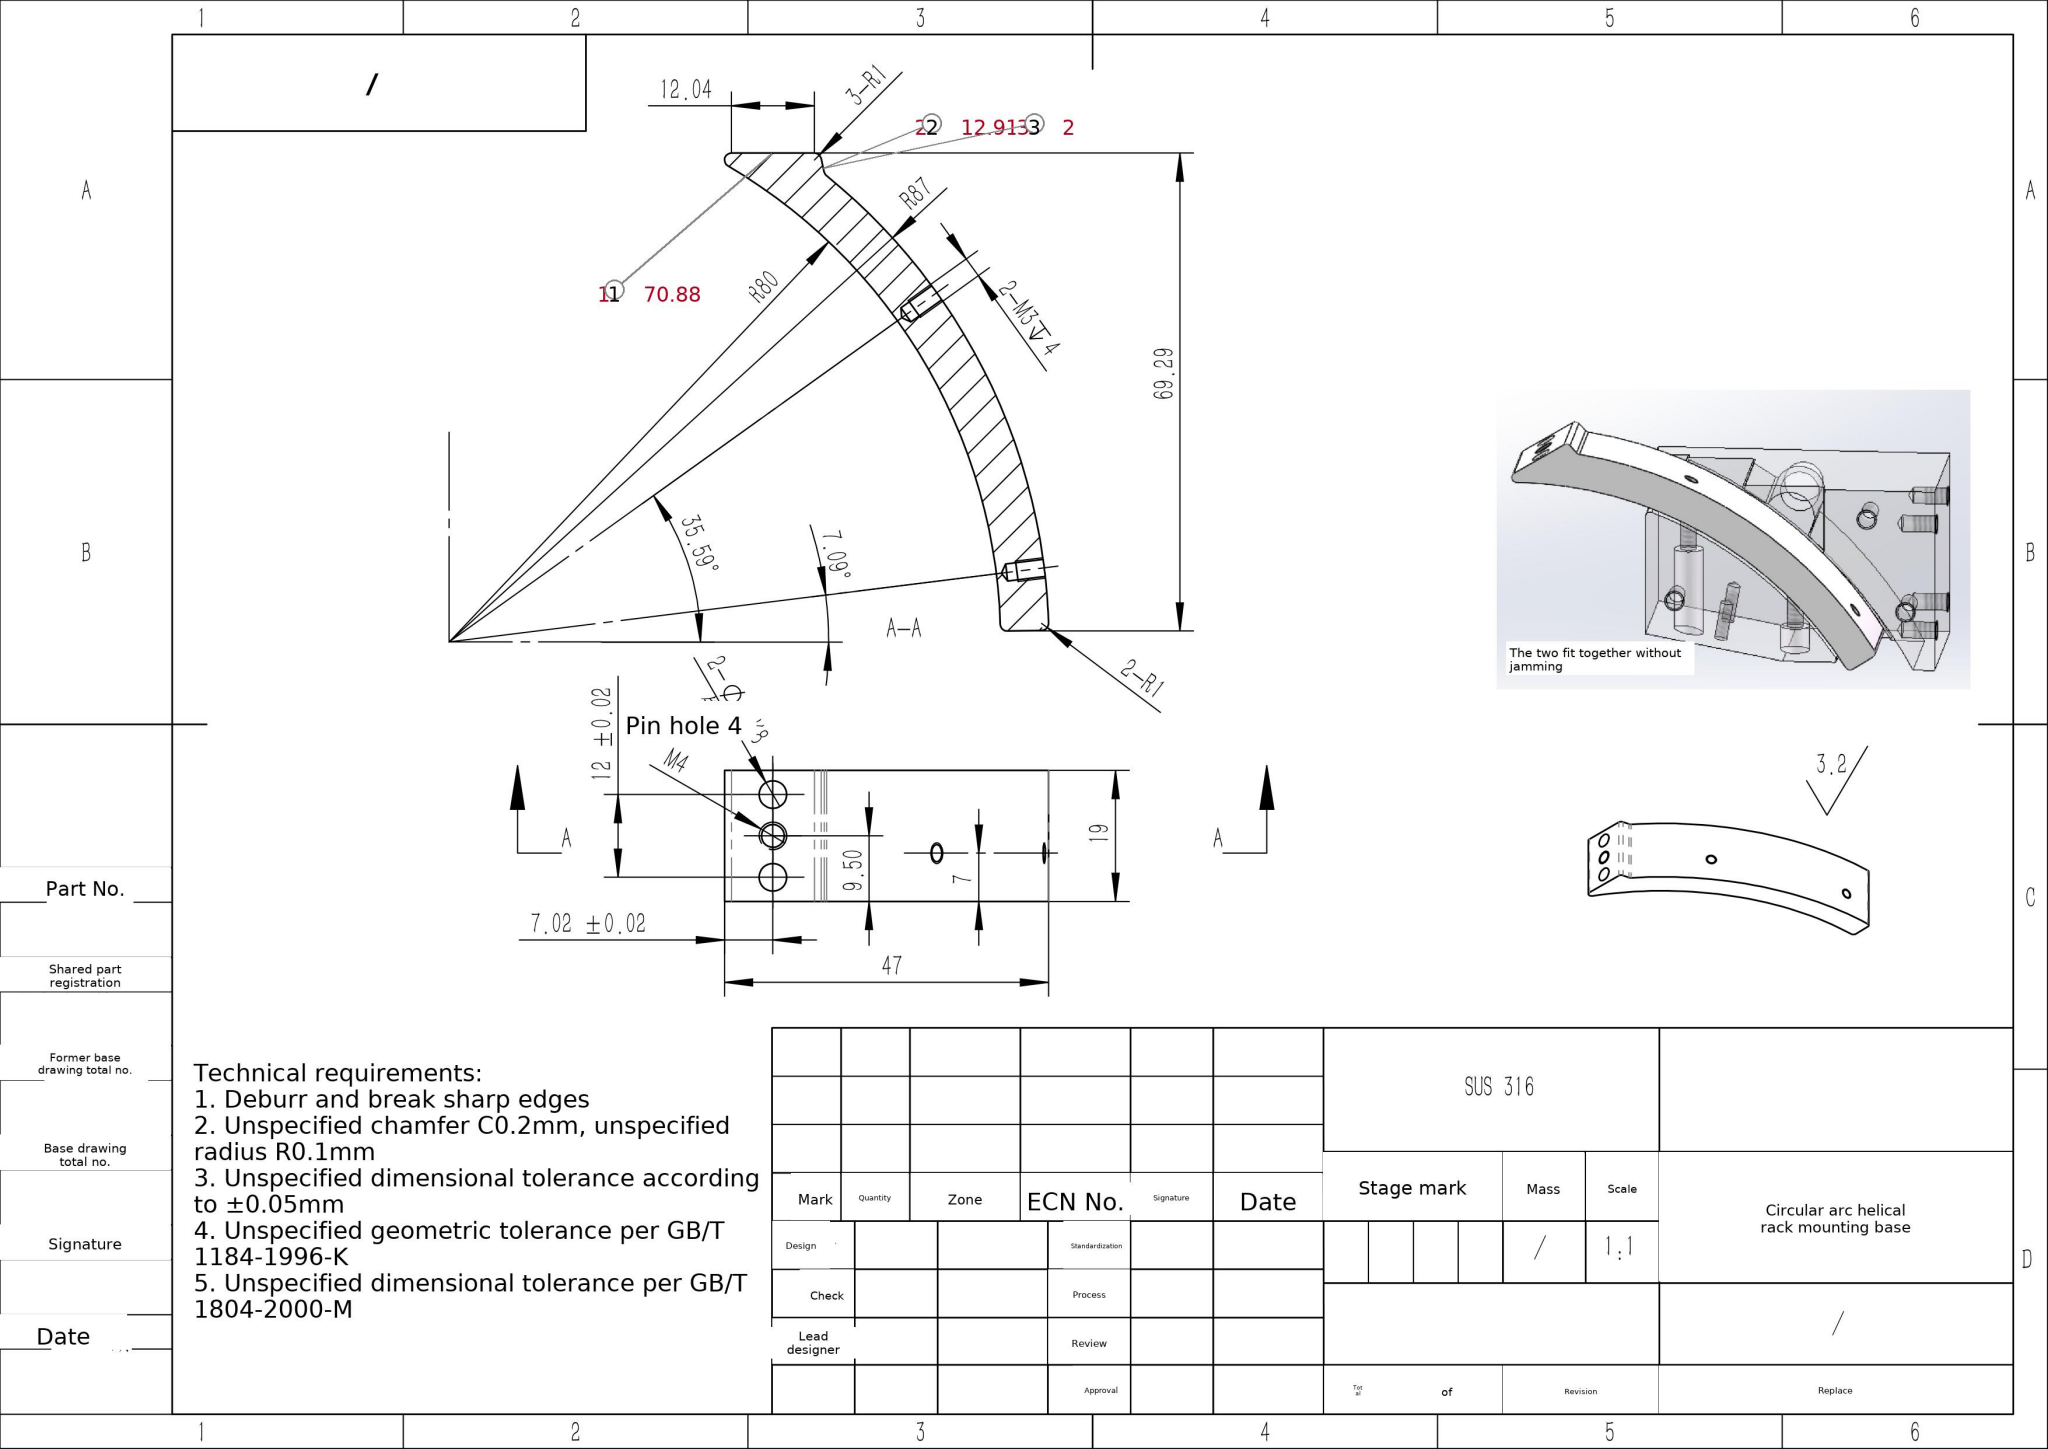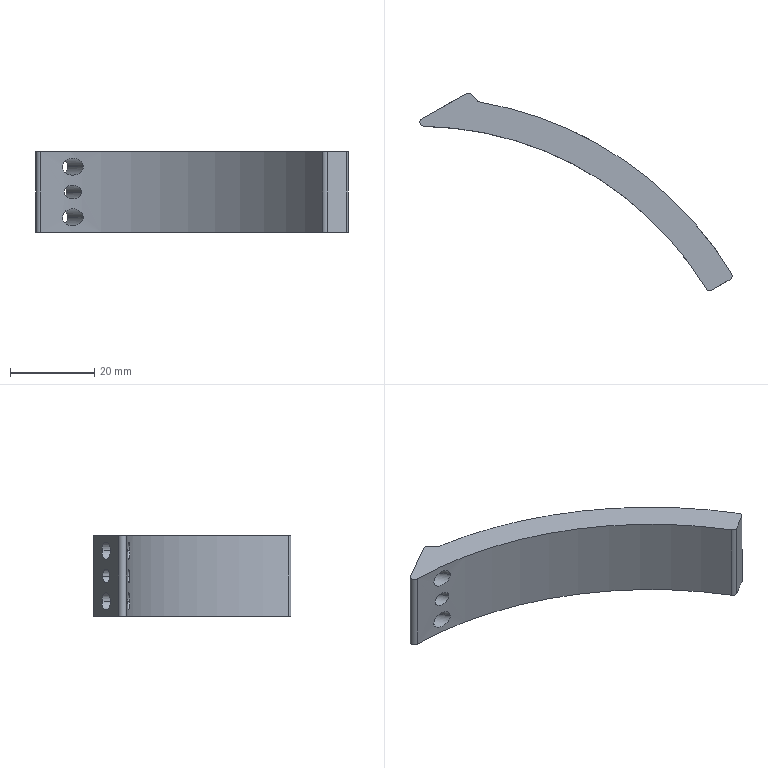Part | SolidWorks | mm | material SUS 316 | 1 solid | 27 faces | box 74.15 x 46.96 x 19 mm | volume 10829 mm3 | cylinder 18 | plane 5 | cone 4 | commonest cylinder face diameters 2 x6 4 x4 2.5 x4 3.3 x2 174 x1 160 x1